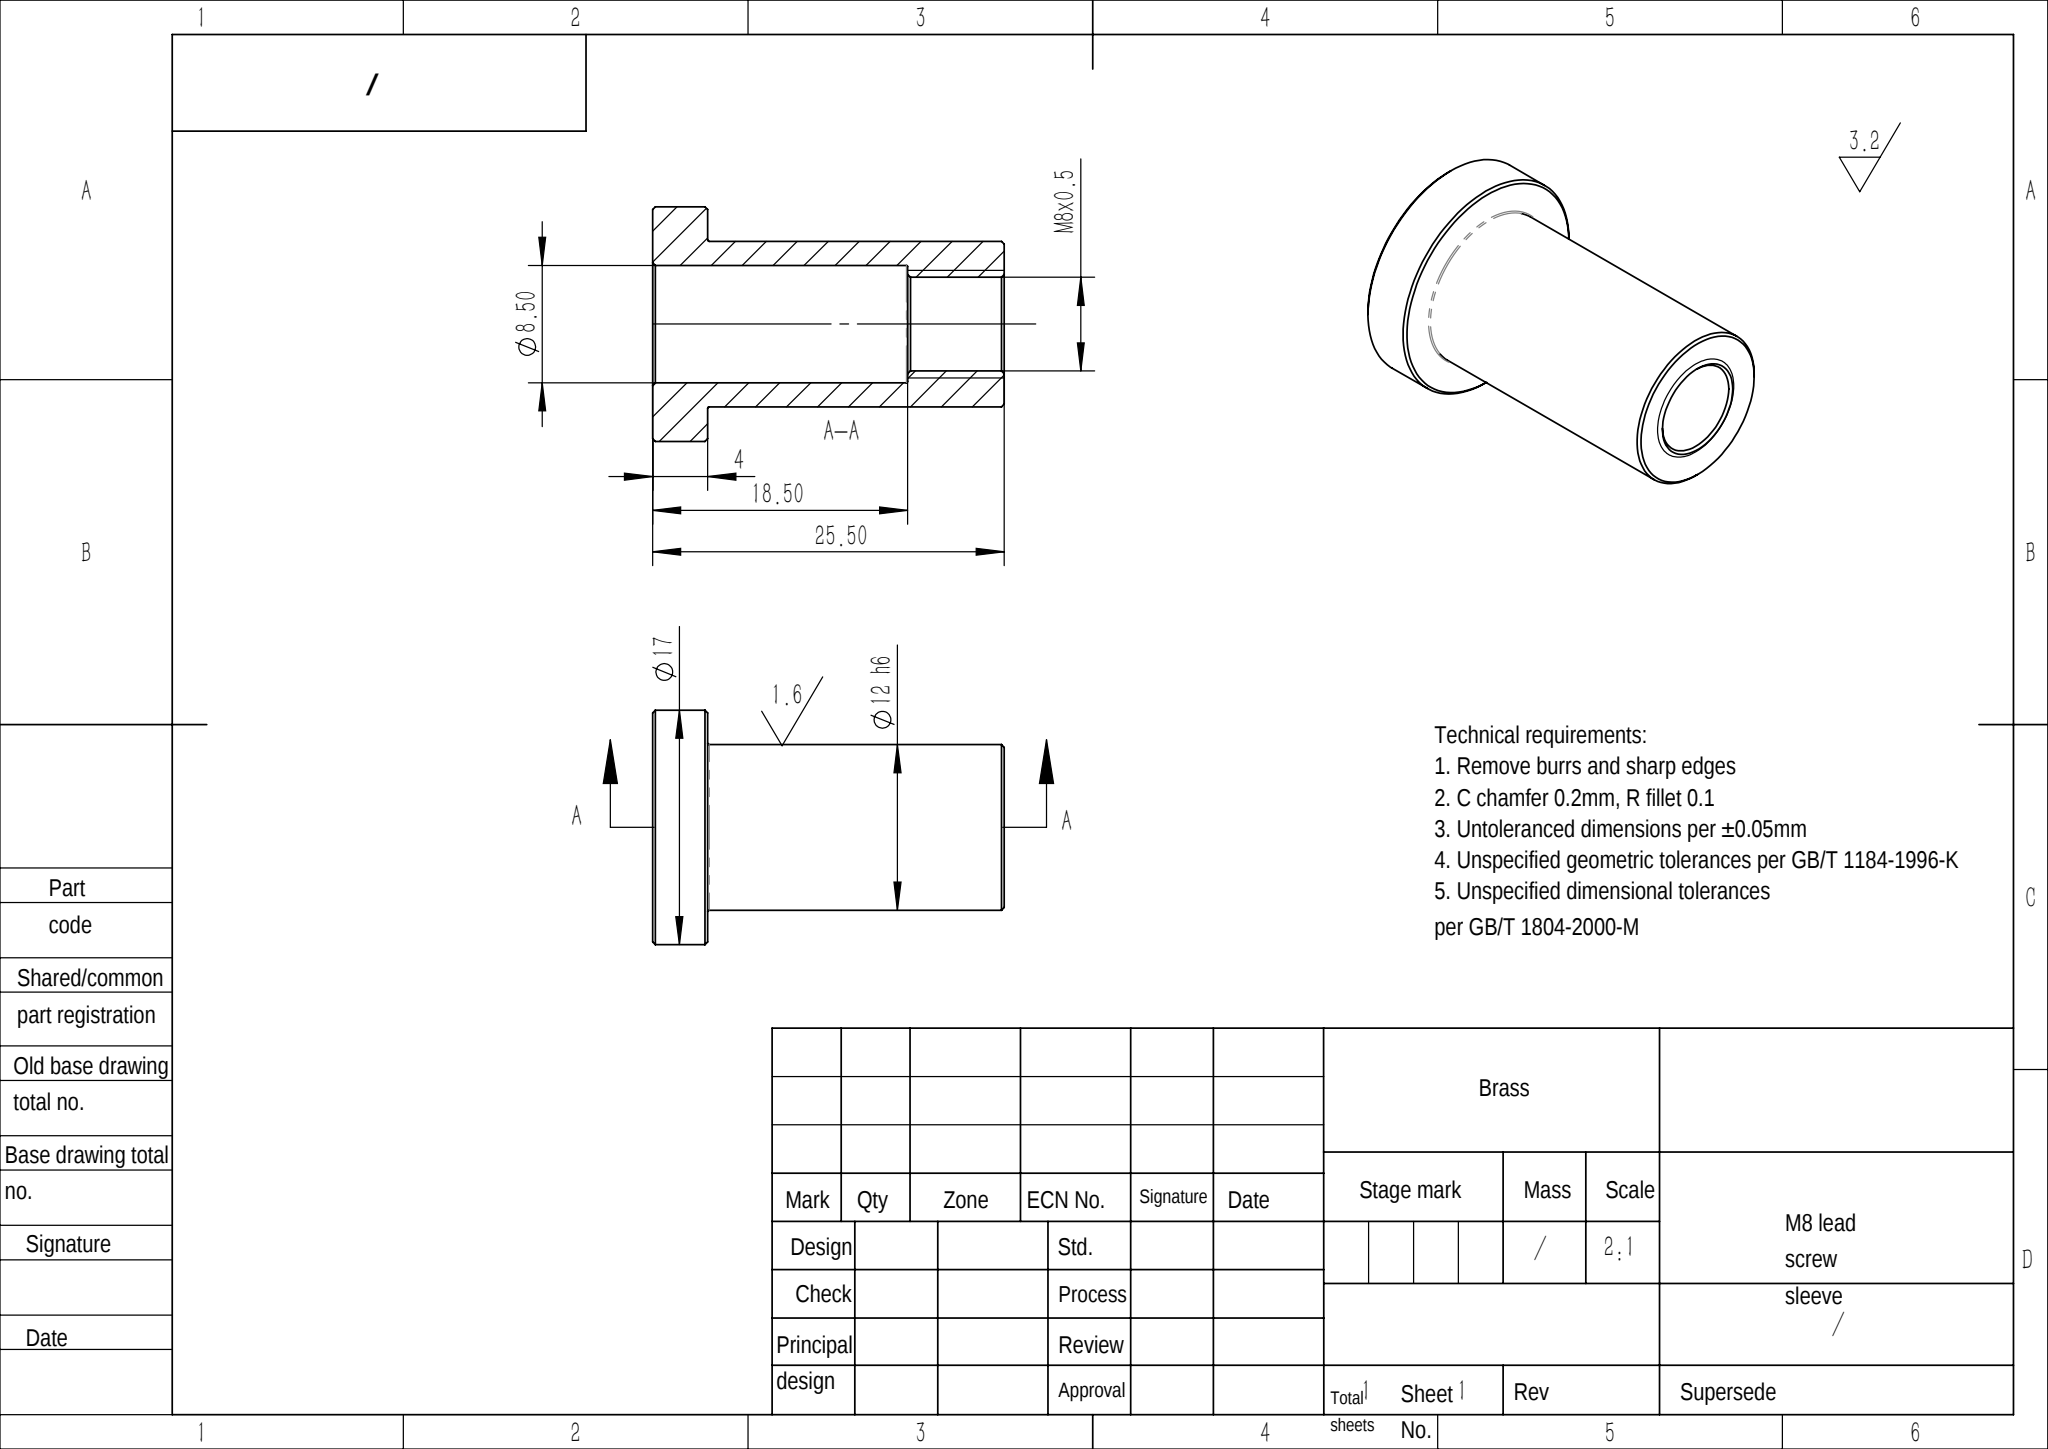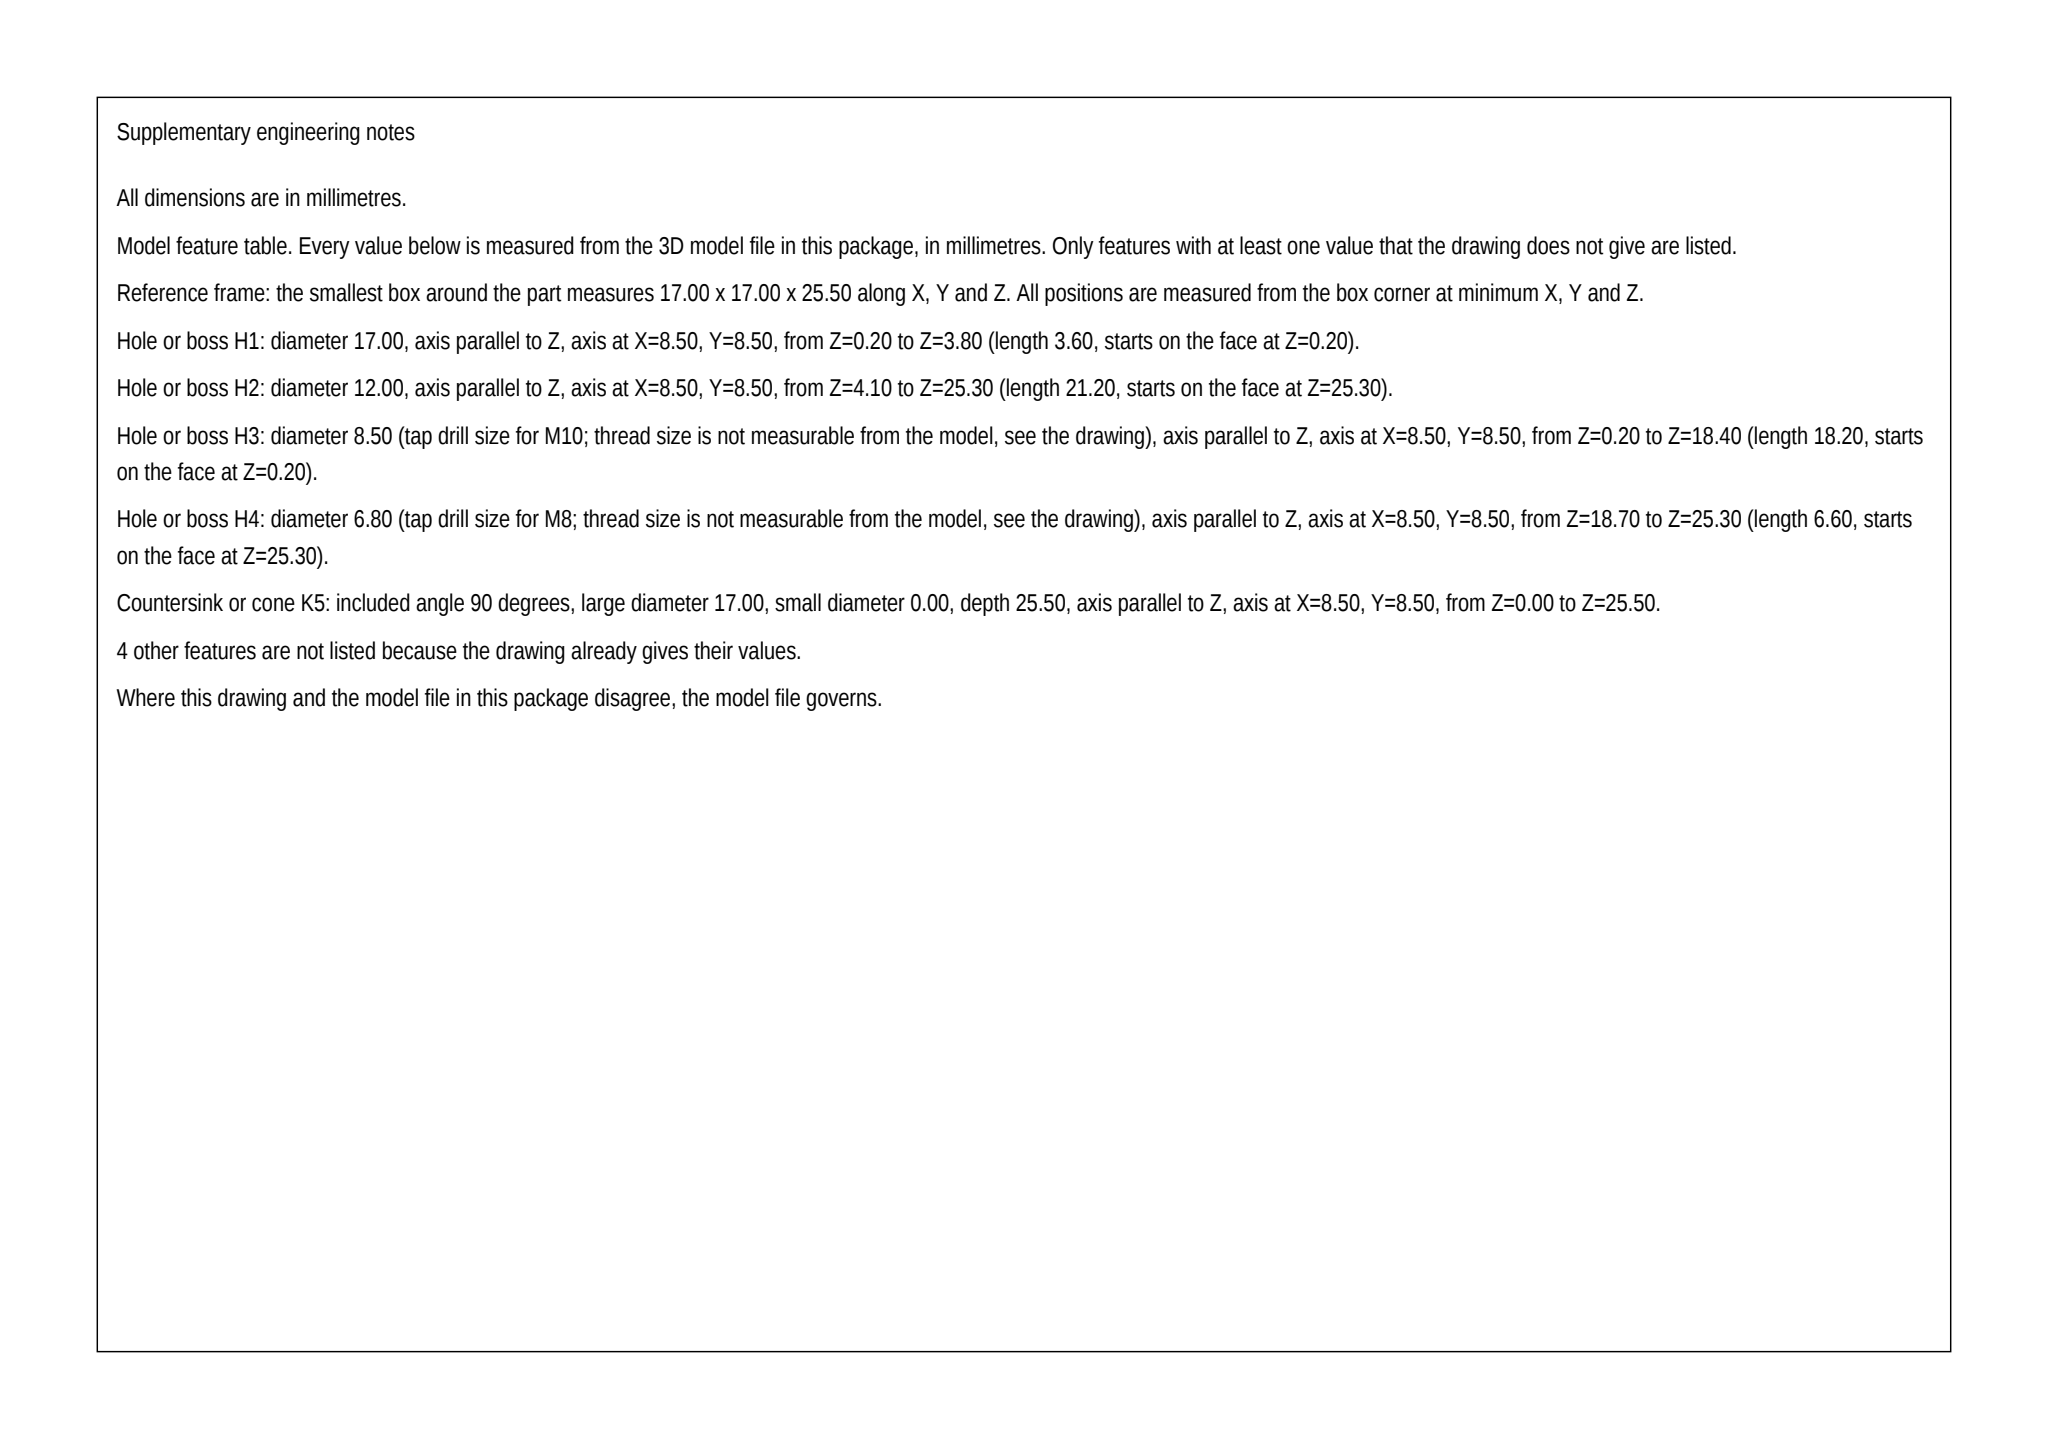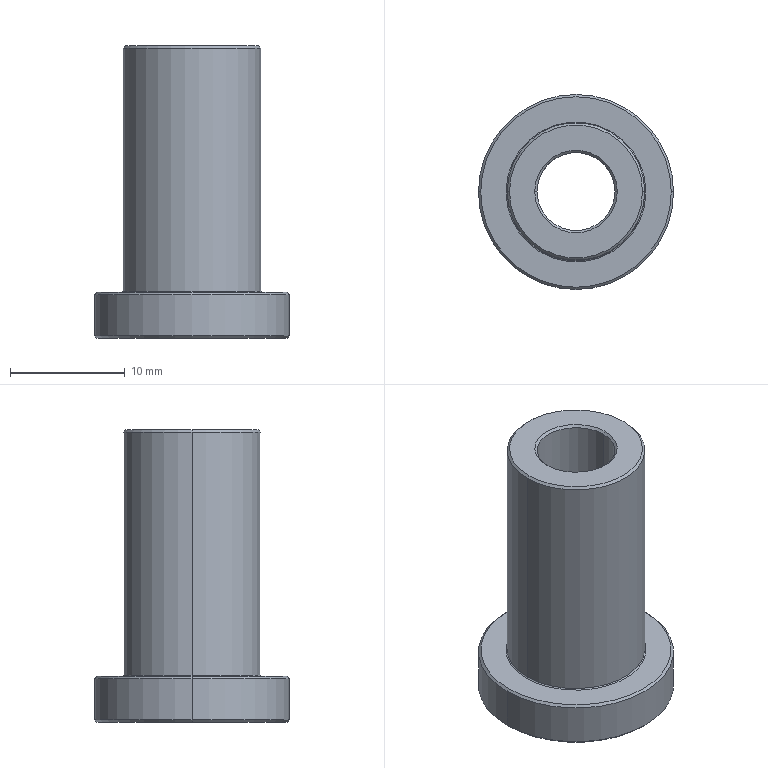Part | SolidWorks | mm | material Brass | 1 solid | 28 faces | box 17 x 17 x 25.5 mm | volume 2031 mm3 | cone 12 | cylinder 8 | torus 4 | plane 4 | commonest cylinder face diameters 6.8 x2 12 x2 8.5 x2 17 x2
STEP:
#1=CARTESIAN_POINT('',(-4.25,0.,18.4));
#2=VERTEX_POINT('',#1);
#3=CARTESIAN_POINT('',(4.25,0.,18.4));
#4=VERTEX_POINT('',#3);
#5=CARTESIAN_POINT('',(0.,0.,18.4));
#6=DIRECTION('',(0.,0.,1.));
#7=DIRECTION('',(1.,0.,0.));
#8=AXIS2_PLACEMENT_3D('',#5,#6,#7);
#9=CIRCLE('',#8,4.25);
#10=EDGE_CURVE('',#2,#4,#9,.T.);
#11=ORIENTED_EDGE('',*,*,#10,.F.);
#12=CARTESIAN_POINT('',(-4.15,0.,18.5));
#13=VERTEX_POINT('',#12);
#14=CARTESIAN_POINT('',(-4.15,0.,18.4));
#15=DIRECTION('',(0.,1.,0.));
#16=DIRECTION('',(-1.,0.,0.));
#17=AXIS2_PLACEMENT_3D('',#14,#15,#16);
#18=CIRCLE('',#17,0.1);
#19=EDGE_CURVE('',#2,#13,#18,.T.);
#20=ORIENTED_EDGE('',*,*,#19,.T.);
#21=CARTESIAN_POINT('',(4.15,0.,18.5));
#22=VERTEX_POINT('',#21);
#23=CARTESIAN_POINT('',(0.,0.,18.5));
#24=DIRECTION('',(0.,0.,-1.));
#25=DIRECTION('',(1.,0.,0.));
#26=AXIS2_PLACEMENT_3D('',#23,#24,#25);
#27=CIRCLE('',#26,4.15);
#28=EDGE_CURVE('',#22,#13,#27,.T.);
#29=ORIENTED_EDGE('',*,*,#28,.F.);
#30=CARTESIAN_POINT('',(4.15,0.,18.4));
#31=DIRECTION('',(0.,-1.,0.));
#32=DIRECTION('',(0.,0.,-1.));
#33=AXIS2_PLACEMENT_3D('',#30,#31,#32);
#34=CIRCLE('',#33,0.1);
#35=EDGE_CURVE('',#4,#22,#34,.T.);
#36=ORIENTED_EDGE('',*,*,#35,.F.);
#37=EDGE_LOOP('',(#11,#20,#29,#36));
#38=FACE_OUTER_BOUND('',#37,.T.);
#39=CARTESIAN_POINT('',(0.,0.,18.4));
#40=DIRECTION('',(0.,0.,1.));
#41=DIRECTION('',(1.,0.,0.));
#42=AXIS2_PLACEMENT_3D('',#39,#40,#41);
#43=TOROIDAL_SURFACE('',#42,4.15,0.1);
#44=ADVANCED_FACE('',(#38),#43,.F.);
#45=CARTESIAN_POINT('',(-6.,0.,4.1));
#46=VERTEX_POINT('',#45);
#47=CARTESIAN_POINT('',(6.,0.,4.1));
#48=VERTEX_POINT('',#47);
#49=CARTESIAN_POINT('',(0.,0.,4.1));
#50=DIRECTION('',(0.,0.,1.));
#51=DIRECTION('',(1.,0.,0.));
#52=AXIS2_PLACEMENT_3D('',#49,#50,#51);
#53=CIRCLE('',#52,6.);
#54=EDGE_CURVE('',#46,#48,#53,.T.);
#55=ORIENTED_EDGE('',*,*,#54,.F.);
#56=CARTESIAN_POINT('',(-6.1,0.,4.));
#57=VERTEX_POINT('',#56);
#58=CARTESIAN_POINT('',(-6.1,0.,4.1));
#59=DIRECTION('',(0.,1.,0.));
#60=DIRECTION('',(-1.,0.,0.));
#61=AXIS2_PLACEMENT_3D('',#58,#59,#60);
#62=CIRCLE('',#61,0.1);
#63=EDGE_CURVE('',#46,#57,#62,.T.);
#64=ORIENTED_EDGE('',*,*,#63,.T.);
#65=CARTESIAN_POINT('',(6.1,0.,4.));
#66=VERTEX_POINT('',#65);
#67=CARTESIAN_POINT('',(0.,0.,4.));
#68=DIRECTION('',(0.,0.,-1.));
#69=DIRECTION('',(1.,0.,0.));
#70=AXIS2_PLACEMENT_3D('',#67,#68,#69);
#71=CIRCLE('',#70,6.1);
#72=EDGE_CURVE('',#66,#57,#71,.T.);
#73=ORIENTED_EDGE('',*,*,#72,.F.);
#74=CARTESIAN_POINT('',(6.1,0.,4.1));
#75=DIRECTION('',(0.,-1.,0.));
#76=DIRECTION('',(0.,0.,-1.));
#77=AXIS2_PLACEMENT_3D('',#74,#75,#76);
#78=CIRCLE('',#77,0.1);
#79=EDGE_CURVE('',#48,#66,#78,.T.);
#80=ORIENTED_EDGE('',*,*,#79,.F.);
#81=EDGE_LOOP('',(#55,#64,#73,#80));
#82=FACE_OUTER_BOUND('',#81,.T.);
#83=CARTESIAN_POINT('',(0.,0.,4.1));
#84=DIRECTION('',(0.,0.,1.));
#85=DIRECTION('',(1.,0.,0.));
#86=AXIS2_PLACEMENT_3D('',#83,#84,#85);
#87=TOROIDAL_SURFACE('',#86,6.1,0.1);
#88=ADVANCED_FACE('',(#82),#87,.F.);
#89=CARTESIAN_POINT('',(8.3,0.,4.));
#90=VERTEX_POINT('',#89);
#91=CARTESIAN_POINT('',(-8.3,0.,4.));
#92=VERTEX_POINT('',#91);
#93=CARTESIAN_POINT('',(0.,0.,4.));
#94=DIRECTION('',(0.,0.,1.));
#95=DIRECTION('',(1.,0.,0.));
#96=AXIS2_PLACEMENT_3D('',#93,#94,#95);
#97=CIRCLE('',#96,8.3);
#98=EDGE_CURVE('',#90,#92,#97,.T.);
#99=ORIENTED_EDGE('',*,*,#98,.F.);
#100=CARTESIAN_POINT('',(8.5,0.,3.8));
#101=VERTEX_POINT('',#100);
#102=CARTESIAN_POINT('',(8.3,0.,4.));
#103=DIRECTION('',(0.7071,0.,-0.7071));
#104=VECTOR('',#103,1000.);
#105=LINE('',#102,#104);
#106=EDGE_CURVE('',#90,#101,#105,.T.);
#107=ORIENTED_EDGE('',*,*,#106,.T.);
#108=CARTESIAN_POINT('',(-8.5,0.,3.8));
#109=VERTEX_POINT('',#108);
#110=CARTESIAN_POINT('',(0.,0.,3.8));
#111=DIRECTION('',(0.,0.,-1.));
#112=DIRECTION('',(1.,0.,0.));
#113=AXIS2_PLACEMENT_3D('',#110,#111,#112);
#114=CIRCLE('',#113,8.5);
#115=EDGE_CURVE('',#109,#101,#114,.T.);
#116=ORIENTED_EDGE('',*,*,#115,.F.);
#117=CARTESIAN_POINT('',(-8.3,0.,4.));
#118=DIRECTION('',(-0.7071,0.,-0.7071));
#119=VECTOR('',#118,1000.);
#120=LINE('',#117,#119);
#121=EDGE_CURVE('',#92,#109,#120,.T.);
#122=ORIENTED_EDGE('',*,*,#121,.F.);
#123=EDGE_LOOP('',(#99,#107,#116,#122));
#124=FACE_OUTER_BOUND('',#123,.T.);
#125=CARTESIAN_POINT('',(0.,0.,4.));
#126=DIRECTION('',(0.,0.,-1.));
#127=DIRECTION('',(-1.,0.,0.));
#128=AXIS2_PLACEMENT_3D('',#125,#126,#127);
#129=CONICAL_SURFACE('',#128,8.3,0.7854);
#130=ADVANCED_FACE('',(#124),#129,.T.);
#131=CARTESIAN_POINT('',(3.4,0.,18.7));
#132=VERTEX_POINT('',#131);
#133=CARTESIAN_POINT('',(-3.4,0.,18.7));
#134=VERTEX_POINT('',#133);
#135=CARTESIAN_POINT('',(0.,0.,18.7));
#136=DIRECTION('',(0.,0.,-1.));
#137=DIRECTION('',(1.,0.,0.));
#138=AXIS2_PLACEMENT_3D('',#135,#136,#137);
#139=CIRCLE('',#138,3.4);
#140=EDGE_CURVE('',#132,#134,#139,.T.);
#141=ORIENTED_EDGE('',*,*,#140,.F.);
#142=CARTESIAN_POINT('',(3.6,0.,18.5));
#143=VERTEX_POINT('',#142);
#144=CARTESIAN_POINT('',(3.6,0.,18.5));
#145=DIRECTION('',(0.7071,0.,-0.7071));
#146=VECTOR('',#145,1000.);
#147=LINE('',#144,#146);
#148=EDGE_CURVE('',#132,#143,#147,.T.);
#149=ORIENTED_EDGE('',*,*,#148,.T.);
#150=CARTESIAN_POINT('',(-3.6,0.,18.5));
#151=VERTEX_POINT('',#150);
#152=CARTESIAN_POINT('',(0.,0.,18.5));
#153=DIRECTION('',(0.,0.,1.));
#154=DIRECTION('',(1.,0.,0.));
#155=AXIS2_PLACEMENT_3D('',#152,#153,#154);
#156=CIRCLE('',#155,3.6);
#157=EDGE_CURVE('',#151,#143,#156,.T.);
#158=ORIENTED_EDGE('',*,*,#157,.F.);
#159=CARTESIAN_POINT('',(-3.6,0.,18.5));
#160=DIRECTION('',(-0.7071,0.,-0.7071));
#161=VECTOR('',#160,1000.);
#162=LINE('',#159,#161);
#163=EDGE_CURVE('',#134,#151,#162,.T.);
#164=ORIENTED_EDGE('',*,*,#163,.F.);
#165=EDGE_LOOP('',(#141,#149,#158,#164));
#166=FACE_OUTER_BOUND('',#165,.T.);
#167=CARTESIAN_POINT('',(0.,0.,18.5));
#168=DIRECTION('',(0.,0.,-1.));
#169=DIRECTION('',(-1.,0.,0.));
#170=AXIS2_PLACEMENT_3D('',#167,#168,#169);
#171=CONICAL_SURFACE('',#170,3.6,0.7854);
#172=ADVANCED_FACE('',(#166),#171,.F.);
#173=CARTESIAN_POINT('',(-8.3,0.,0.));
#174=VERTEX_POINT('',#173);
#175=CARTESIAN_POINT('',(8.3,0.,0.));
#176=VERTEX_POINT('',#175);
#177=CARTESIAN_POINT('',(0.,0.,0.));
#178=DIRECTION('',(0.,0.,-1.));
#179=DIRECTION('',(1.,0.,0.));
#180=AXIS2_PLACEMENT_3D('',#177,#178,#179);
#181=CIRCLE('',#180,8.3);
#182=EDGE_CURVE('',#174,#176,#181,.T.);
#183=ORIENTED_EDGE('',*,*,#182,.F.);
#184=CARTESIAN_POINT('',(-8.5,0.,0.2));
#185=VERTEX_POINT('',#184);
#186=CARTESIAN_POINT('',(-8.5,0.,0.2));
#187=DIRECTION('',(-0.7071,0.,0.7071));
#188=VECTOR('',#187,1000.);
#189=LINE('',#186,#188);
#190=EDGE_CURVE('',#174,#185,#189,.T.);
#191=ORIENTED_EDGE('',*,*,#190,.T.);
#192=CARTESIAN_POINT('',(8.5,0.,0.2));
#193=VERTEX_POINT('',#192);
#194=CARTESIAN_POINT('',(0.,0.,0.2));
#195=DIRECTION('',(0.,0.,1.));
#196=DIRECTION('',(1.,0.,0.));
#197=AXIS2_PLACEMENT_3D('',#194,#195,#196);
#198=CIRCLE('',#197,8.5);
#199=EDGE_CURVE('',#193,#185,#198,.T.);
#200=ORIENTED_EDGE('',*,*,#199,.F.);
#201=CARTESIAN_POINT('',(8.5,0.,0.2));
#202=DIRECTION('',(0.7071,0.,0.7071));
#203=VECTOR('',#202,1000.);
#204=LINE('',#201,#203);
#205=EDGE_CURVE('',#176,#193,#204,.T.);
#206=ORIENTED_EDGE('',*,*,#205,.F.);
#207=EDGE_LOOP('',(#183,#191,#200,#206));
#208=FACE_OUTER_BOUND('',#207,.T.);
#209=CARTESIAN_POINT('',(0.,0.,0.2));
#210=DIRECTION('',(0.,0.,1.));
#211=DIRECTION('',(1.,0.,0.));
#212=AXIS2_PLACEMENT_3D('',#209,#210,#211);
#213=CONICAL_SURFACE('',#212,8.5,0.7854);
#214=ADVANCED_FACE('',(#208),#213,.T.);
#215=CARTESIAN_POINT('',(4.25,0.,0.2));
#216=VERTEX_POINT('',#215);
#217=CARTESIAN_POINT('',(-4.25,0.,0.2));
#218=VERTEX_POINT('',#217);
#219=CARTESIAN_POINT('',(0.,0.,0.2));
#220=DIRECTION('',(0.,0.,-1.));
#221=DIRECTION('',(1.,0.,0.));
#222=AXIS2_PLACEMENT_3D('',#219,#220,#221);
#223=CIRCLE('',#222,4.25);
#224=EDGE_CURVE('',#216,#218,#223,.T.);
#225=ORIENTED_EDGE('',*,*,#224,.F.);
#226=CARTESIAN_POINT('',(4.45,0.,0.));
#227=VERTEX_POINT('',#226);
#228=CARTESIAN_POINT('',(4.45,0.,0.));
#229=DIRECTION('',(0.7071,0.,-0.7071));
#230=VECTOR('',#229,1000.);
#231=LINE('',#228,#230);
#232=EDGE_CURVE('',#216,#227,#231,.T.);
#233=ORIENTED_EDGE('',*,*,#232,.T.);
#234=CARTESIAN_POINT('',(-4.45,0.,0.));
#235=VERTEX_POINT('',#234);
#236=CARTESIAN_POINT('',(0.,0.,0.));
#237=DIRECTION('',(0.,0.,1.));
#238=DIRECTION('',(1.,0.,0.));
#239=AXIS2_PLACEMENT_3D('',#236,#237,#238);
#240=CIRCLE('',#239,4.45);
#241=EDGE_CURVE('',#235,#227,#240,.T.);
#242=ORIENTED_EDGE('',*,*,#241,.F.);
#243=CARTESIAN_POINT('',(-4.45,0.,0.));
#244=DIRECTION('',(-0.7071,0.,-0.7071));
#245=VECTOR('',#244,1000.);
#246=LINE('',#243,#245);
#247=EDGE_CURVE('',#218,#235,#246,.T.);
#248=ORIENTED_EDGE('',*,*,#247,.F.);
#249=EDGE_LOOP('',(#225,#233,#242,#248));
#250=FACE_OUTER_BOUND('',#249,.T.);
#251=CARTESIAN_POINT('',(0.,0.,0.));
#252=DIRECTION('',(0.,0.,-1.));
#253=DIRECTION('',(-1.,0.,0.));
#254=AXIS2_PLACEMENT_3D('',#251,#252,#253);
#255=CONICAL_SURFACE('',#254,4.45,0.7854);
#256=ADVANCED_FACE('',(#250),#255,.F.);
#257=CARTESIAN_POINT('',(5.8,0.,25.5));
#258=VERTEX_POINT('',#257);
#259=CARTESIAN_POINT('',(-5.8,0.,25.5));
#260=VERTEX_POINT('',#259);
#261=CARTESIAN_POINT('',(0.,0.,25.5));
#262=DIRECTION('',(0.,0.,1.));
#263=DIRECTION('',(1.,0.,0.));
#264=AXIS2_PLACEMENT_3D('',#261,#262,#263);
#265=CIRCLE('',#264,5.8);
#266=EDGE_CURVE('',#258,#260,#265,.T.);
#267=ORIENTED_EDGE('',*,*,#266,.F.);
#268=CARTESIAN_POINT('',(6.,0.,25.3));
#269=VERTEX_POINT('',#268);
#270=CARTESIAN_POINT('',(5.8,0.,25.5));
#271=DIRECTION('',(0.7071,0.,-0.7071));
#272=VECTOR('',#271,1000.);
#273=LINE('',#270,#272);
#274=EDGE_CURVE('',#258,#269,#273,.T.);
#275=ORIENTED_EDGE('',*,*,#274,.T.);
#276=CARTESIAN_POINT('',(-6.,0.,25.3));
#277=VERTEX_POINT('',#276);
#278=CARTESIAN_POINT('',(0.,0.,25.3));
#279=DIRECTION('',(0.,0.,-1.));
#280=DIRECTION('',(1.,0.,0.));
#281=AXIS2_PLACEMENT_3D('',#278,#279,#280);
#282=CIRCLE('',#281,6.);
#283=EDGE_CURVE('',#277,#269,#282,.T.);
#284=ORIENTED_EDGE('',*,*,#283,.F.);
#285=CARTESIAN_POINT('',(-5.8,0.,25.5));
#286=DIRECTION('',(-0.7071,0.,-0.7071));
#287=VECTOR('',#286,1000.);
#288=LINE('',#285,#287);
#289=EDGE_CURVE('',#260,#277,#288,.T.);
#290=ORIENTED_EDGE('',*,*,#289,.F.);
#291=EDGE_LOOP('',(#267,#275,#284,#290));
#292=FACE_OUTER_BOUND('',#291,.T.);
#293=CARTESIAN_POINT('',(0.,0.,25.5));
#294=DIRECTION('',(0.,0.,-1.));
#295=DIRECTION('',(-1.,0.,0.));
#296=AXIS2_PLACEMENT_3D('',#293,#294,#295);
#297=CONICAL_SURFACE('',#296,5.8,0.7854);
#298=ADVANCED_FACE('',(#292),#297,.T.);
#299=CARTESIAN_POINT('',(-3.4,0.,25.3));
#300=VERTEX_POINT('',#299);
#301=CARTESIAN_POINT('',(3.4,0.,25.3));
#302=VERTEX_POINT('',#301);
#303=CARTESIAN_POINT('',(0.,0.,25.3));
#304=DIRECTION('',(0.,0.,1.));
#305=DIRECTION('',(1.,0.,0.));
#306=AXIS2_PLACEMENT_3D('',#303,#304,#305);
#307=CIRCLE('',#306,3.4);
#308=EDGE_CURVE('',#300,#302,#307,.T.);
#309=ORIENTED_EDGE('',*,*,#308,.F.);
#310=CARTESIAN_POINT('',(-3.6,0.,25.5));
#311=VERTEX_POINT('',#310);
#312=CARTESIAN_POINT('',(-3.4,0.,25.3));
#313=DIRECTION('',(-0.7071,0.,0.7071));
#314=VECTOR('',#313,1000.);
#315=LINE('',#312,#314);
#316=EDGE_CURVE('',#300,#311,#315,.T.);
#317=ORIENTED_EDGE('',*,*,#316,.T.);
#318=CARTESIAN_POINT('',(3.6,0.,25.5));
#319=VERTEX_POINT('',#318);
#320=CARTESIAN_POINT('',(0.,0.,25.5));
#321=DIRECTION('',(0.,0.,-1.));
#322=DIRECTION('',(1.,0.,0.));
#323=AXIS2_PLACEMENT_3D('',#320,#321,#322);
#324=CIRCLE('',#323,3.6);
#325=EDGE_CURVE('',#319,#311,#324,.T.);
#326=ORIENTED_EDGE('',*,*,#325,.F.);
#327=CARTESIAN_POINT('',(3.4,0.,25.3));
#328=DIRECTION('',(0.7071,0.,0.7071));
#329=VECTOR('',#328,1000.);
#330=LINE('',#327,#329);
#331=EDGE_CURVE('',#302,#319,#330,.T.);
#332=ORIENTED_EDGE('',*,*,#331,.F.);
#333=EDGE_LOOP('',(#309,#317,#326,#332));
#334=FACE_OUTER_BOUND('',#333,.T.);
#335=CARTESIAN_POINT('',(0.,0.,25.3));
#336=DIRECTION('',(0.,0.,1.));
#337=DIRECTION('',(1.,0.,0.));
#338=AXIS2_PLACEMENT_3D('',#335,#336,#337);
#339=CONICAL_SURFACE('',#338,3.4,0.7854);
#340=ADVANCED_FACE('',(#334),#339,.F.);
#341=ORIENTED_EDGE('',*,*,#308,.T.);
#342=CARTESIAN_POINT('',(3.4,0.,30.));
#343=DIRECTION('',(0.,0.,-1.));
#344=VECTOR('',#343,1000.);
#345=LINE('',#342,#344);
#346=EDGE_CURVE('',#302,#132,#345,.T.);
#347=ORIENTED_EDGE('',*,*,#346,.T.);
#348=ORIENTED_EDGE('',*,*,#140,.T.);
#349=CARTESIAN_POINT('',(-3.4,0.,30.));
#350=DIRECTION('',(0.,0.,-1.));
#351=VECTOR('',#350,1000.);
#352=LINE('',#349,#351);
#353=EDGE_CURVE('',#300,#134,#352,.T.);
#354=ORIENTED_EDGE('',*,*,#353,.F.);
#355=EDGE_LOOP('',(#341,#347,#348,#354));
#356=FACE_OUTER_BOUND('',#355,.T.);
#357=CARTESIAN_POINT('',(0.,0.,30.));
#358=DIRECTION('',(0.,0.,-1.));
#359=DIRECTION('',(-1.,0.,0.));
#360=AXIS2_PLACEMENT_3D('',#357,#358,#359);
#361=CYLINDRICAL_SURFACE('',#360,3.4);
#362=ADVANCED_FACE('',(#356),#361,.F.);
#363=CARTESIAN_POINT('',(0.,0.,4.1));
#364=DIRECTION('',(0.,0.,1.));
#365=DIRECTION('',(1.,0.,0.));
#366=AXIS2_PLACEMENT_3D('',#363,#364,#365);
#367=CIRCLE('',#366,6.);
#368=EDGE_CURVE('',#48,#46,#367,.T.);
#369=ORIENTED_EDGE('',*,*,#368,.T.);
#370=CARTESIAN_POINT('',(-6.,0.,4.));
#371=DIRECTION('',(0.,0.,1.));
#372=VECTOR('',#371,1000.);
#373=LINE('',#370,#372);
#374=EDGE_CURVE('',#46,#277,#373,.T.);
#375=ORIENTED_EDGE('',*,*,#374,.T.);
#376=ORIENTED_EDGE('',*,*,#283,.T.);
#377=CARTESIAN_POINT('',(6.,0.,4.));
#378=DIRECTION('',(0.,0.,1.));
#379=VECTOR('',#378,1000.);
#380=LINE('',#377,#379);
#381=EDGE_CURVE('',#48,#269,#380,.T.);
#382=ORIENTED_EDGE('',*,*,#381,.F.);
#383=EDGE_LOOP('',(#369,#375,#376,#382));
#384=FACE_OUTER_BOUND('',#383,.T.);
#385=CARTESIAN_POINT('',(0.,0.,4.));
#386=DIRECTION('',(0.,0.,1.));
#387=DIRECTION('',(1.,0.,0.));
#388=AXIS2_PLACEMENT_3D('',#385,#386,#387);
#389=CYLINDRICAL_SURFACE('',#388,6.);
#390=ADVANCED_FACE('',(#384),#389,.T.);
#391=ORIENTED_EDGE('',*,*,#10,.T.);
#392=CARTESIAN_POINT('',(4.25,0.,18.5));
#393=DIRECTION('',(0.,0.,-1.));
#394=VECTOR('',#393,1000.);
#395=LINE('',#392,#394);
#396=EDGE_CURVE('',#4,#216,#395,.T.);
#397=ORIENTED_EDGE('',*,*,#396,.T.);
#398=ORIENTED_EDGE('',*,*,#224,.T.);
#399=CARTESIAN_POINT('',(-4.25,0.,18.5));
#400=DIRECTION('',(0.,0.,-1.));
#401=VECTOR('',#400,1000.);
#402=LINE('',#399,#401);
#403=EDGE_CURVE('',#2,#218,#402,.T.);
#404=ORIENTED_EDGE('',*,*,#403,.F.);
#405=EDGE_LOOP('',(#391,#397,#398,#404));
#406=FACE_OUTER_BOUND('',#405,.T.);
#407=CARTESIAN_POINT('',(0.,0.,18.5));
#408=DIRECTION('',(0.,0.,-1.));
#409=DIRECTION('',(-1.,0.,0.));
#410=AXIS2_PLACEMENT_3D('',#407,#408,#409);
#411=CYLINDRICAL_SURFACE('',#410,4.25);
#412=ADVANCED_FACE('',(#406),#411,.F.);
#413=ORIENTED_EDGE('',*,*,#115,.T.);
#414=CARTESIAN_POINT('',(8.5,0.,18.5));
#415=DIRECTION('',(0.,0.,-1.));
#416=VECTOR('',#415,1000.);
#417=LINE('',#414,#416);
#418=EDGE_CURVE('',#101,#193,#417,.T.);
#419=ORIENTED_EDGE('',*,*,#418,.T.);
#420=ORIENTED_EDGE('',*,*,#199,.T.);
#421=CARTESIAN_POINT('',(-8.5,0.,18.5));
#422=DIRECTION('',(0.,0.,-1.));
#423=VECTOR('',#422,1000.);
#424=LINE('',#421,#423);
#425=EDGE_CURVE('',#109,#185,#424,.T.);
#426=ORIENTED_EDGE('',*,*,#425,.F.);
#427=EDGE_LOOP('',(#413,#419,#420,#426));
#428=FACE_OUTER_BOUND('',#427,.T.);
#429=CARTESIAN_POINT('',(0.,0.,18.5));
#430=DIRECTION('',(0.,0.,-1.));
#431=DIRECTION('',(-1.,0.,0.));
#432=AXIS2_PLACEMENT_3D('',#429,#430,#431);
#433=CYLINDRICAL_SURFACE('',#432,8.5);
#434=ADVANCED_FACE('',(#428),#433,.T.);
#435=ORIENTED_EDGE('',*,*,#418,.F.);
#436=CARTESIAN_POINT('',(0.,0.,3.8));
#437=DIRECTION('',(0.,0.,-1.));
#438=DIRECTION('',(1.,0.,0.));
#439=AXIS2_PLACEMENT_3D('',#436,#437,#438);
#440=CIRCLE('',#439,8.5);
#441=EDGE_CURVE('',#101,#109,#440,.T.);
#442=ORIENTED_EDGE('',*,*,#441,.T.);
#443=ORIENTED_EDGE('',*,*,#425,.T.);
#444=CARTESIAN_POINT('',(0.,0.,0.2));
#445=DIRECTION('',(0.,0.,1.));
#446=DIRECTION('',(1.,0.,0.));
#447=AXIS2_PLACEMENT_3D('',#444,#445,#446);
#448=CIRCLE('',#447,8.5);
#449=EDGE_CURVE('',#185,#193,#448,.T.);
#450=ORIENTED_EDGE('',*,*,#449,.T.);
#451=EDGE_LOOP('',(#435,#442,#443,#450));
#452=FACE_OUTER_BOUND('',#451,.T.);
#453=CARTESIAN_POINT('',(0.,0.,18.5));
#454=DIRECTION('',(0.,0.,-1.));
#455=DIRECTION('',(-1.,0.,0.));
#456=AXIS2_PLACEMENT_3D('',#453,#454,#455);
#457=CYLINDRICAL_SURFACE('',#456,8.5);
#458=ADVANCED_FACE('',(#452),#457,.T.);
#459=ORIENTED_EDGE('',*,*,#241,.T.);
#460=CARTESIAN_POINT('',(0.,0.,0.));
#461=DIRECTION('',(0.,0.,1.));
#462=DIRECTION('',(1.,0.,0.));
#463=AXIS2_PLACEMENT_3D('',#460,#461,#462);
#464=CIRCLE('',#463,4.45);
#465=EDGE_CURVE('',#227,#235,#464,.T.);
#466=ORIENTED_EDGE('',*,*,#465,.T.);
#467=EDGE_LOOP('',(#459,#466));
#468=FACE_BOUND('',#467,.T.);
#469=CARTESIAN_POINT('',(0.,0.,0.));
#470=DIRECTION('',(0.,0.,-1.));
#471=DIRECTION('',(1.,0.,0.));
#472=AXIS2_PLACEMENT_3D('',#469,#470,#471);
#473=CIRCLE('',#472,8.3);
#474=EDGE_CURVE('',#176,#174,#473,.T.);
#475=ORIENTED_EDGE('',*,*,#474,.T.);
#476=ORIENTED_EDGE('',*,*,#182,.T.);
#477=EDGE_LOOP('',(#475,#476));
#478=FACE_OUTER_BOUND('',#477,.T.);
#479=CARTESIAN_POINT('',(0.,0.,0.));
#480=DIRECTION('',(0.,0.,1.));
#481=DIRECTION('',(1.,0.,0.));
#482=AXIS2_PLACEMENT_3D('',#479,#480,#481);
#483=PLANE('',#482);
#484=ADVANCED_FACE('',(#468,#478),#483,.F.);
#485=ORIENTED_EDGE('',*,*,#396,.F.);
#486=CARTESIAN_POINT('',(0.,0.,18.4));
#487=DIRECTION('',(0.,0.,1.));
#488=DIRECTION('',(1.,0.,0.));
#489=AXIS2_PLACEMENT_3D('',#486,#487,#488);
#490=CIRCLE('',#489,4.25);
#491=EDGE_CURVE('',#4,#2,#490,.T.);
#492=ORIENTED_EDGE('',*,*,#491,.T.);
#493=ORIENTED_EDGE('',*,*,#403,.T.);
#494=CARTESIAN_POINT('',(0.,0.,0.2));
#495=DIRECTION('',(0.,0.,-1.));
#496=DIRECTION('',(1.,0.,0.));
#497=AXIS2_PLACEMENT_3D('',#494,#495,#496);
#498=CIRCLE('',#497,4.25);
#499=EDGE_CURVE('',#218,#216,#498,.T.);
#500=ORIENTED_EDGE('',*,*,#499,.T.);
#501=EDGE_LOOP('',(#485,#492,#493,#500));
#502=FACE_OUTER_BOUND('',#501,.T.);
#503=CARTESIAN_POINT('',(0.,0.,18.5));
#504=DIRECTION('',(0.,0.,-1.));
#505=DIRECTION('',(-1.,0.,0.));
#506=AXIS2_PLACEMENT_3D('',#503,#504,#505);
#507=CYLINDRICAL_SURFACE('',#506,4.25);
#508=ADVANCED_FACE('',(#502),#507,.F.);
#509=ORIENTED_EDGE('',*,*,#72,.T.);
#510=CARTESIAN_POINT('',(0.,0.,4.));
#511=DIRECTION('',(0.,0.,-1.));
#512=DIRECTION('',(1.,0.,0.));
#513=AXIS2_PLACEMENT_3D('',#510,#511,#512);
#514=CIRCLE('',#513,6.1);
#515=EDGE_CURVE('',#57,#66,#514,.T.);
#516=ORIENTED_EDGE('',*,*,#515,.T.);
#517=EDGE_LOOP('',(#509,#516));
#518=FACE_BOUND('',#517,.T.);
#519=CARTESIAN_POINT('',(0.,0.,4.));
#520=DIRECTION('',(0.,0.,1.));
#521=DIRECTION('',(1.,0.,0.));
#522=AXIS2_PLACEMENT_3D('',#519,#520,#521);
#523=CIRCLE('',#522,8.3);
#524=EDGE_CURVE('',#92,#90,#523,.T.);
#525=ORIENTED_EDGE('',*,*,#524,.T.);
#526=ORIENTED_EDGE('',*,*,#98,.T.);
#527=EDGE_LOOP('',(#525,#526));
#528=FACE_OUTER_BOUND('',#527,.T.);
#529=CARTESIAN_POINT('',(0.,0.,4.));
#530=DIRECTION('',(0.,0.,1.));
#531=DIRECTION('',(1.,0.,0.));
#532=AXIS2_PLACEMENT_3D('',#529,#530,#531);
#533=PLANE('',#532);
#534=ADVANCED_FACE('',(#518,#528),#533,.T.);
#535=ORIENTED_EDGE('',*,*,#374,.F.);
#536=ORIENTED_EDGE('',*,*,#54,.T.);
#537=ORIENTED_EDGE('',*,*,#381,.T.);
#538=CARTESIAN_POINT('',(0.,0.,25.3));
#539=DIRECTION('',(0.,0.,-1.));
#540=DIRECTION('',(1.,0.,0.));
#541=AXIS2_PLACEMENT_3D('',#538,#539,#540);
#542=CIRCLE('',#541,6.);
#543=EDGE_CURVE('',#269,#277,#542,.T.);
#544=ORIENTED_EDGE('',*,*,#543,.T.);
#545=EDGE_LOOP('',(#535,#536,#537,#544));
#546=FACE_OUTER_BOUND('',#545,.T.);
#547=CARTESIAN_POINT('',(0.,0.,4.));
#548=DIRECTION('',(0.,0.,1.));
#549=DIRECTION('',(1.,0.,0.));
#550=AXIS2_PLACEMENT_3D('',#547,#548,#549);
#551=CYLINDRICAL_SURFACE('',#550,6.);
#552=ADVANCED_FACE('',(#546),#551,.T.);
#553=ORIENTED_EDGE('',*,*,#28,.T.);
#554=CARTESIAN_POINT('',(0.,0.,18.5));
#555=DIRECTION('',(0.,0.,-1.));
#556=DIRECTION('',(1.,0.,0.));
#557=AXIS2_PLACEMENT_3D('',#554,#555,#556);
#558=CIRCLE('',#557,4.15);
#559=EDGE_CURVE('',#13,#22,#558,.T.);
#560=ORIENTED_EDGE('',*,*,#559,.T.);
#561=EDGE_LOOP('',(#553,#560));
#562=FACE_OUTER_BOUND('',#561,.T.);
#563=ORIENTED_EDGE('',*,*,#157,.T.);
#564=CARTESIAN_POINT('',(0.,0.,18.5));
#565=DIRECTION('',(0.,0.,1.));
#566=DIRECTION('',(1.,0.,0.));
#567=AXIS2_PLACEMENT_3D('',#564,#565,#566);
#568=CIRCLE('',#567,3.6);
#569=EDGE_CURVE('',#143,#151,#568,.T.);
#570=ORIENTED_EDGE('',*,*,#569,.T.);
#571=EDGE_LOOP('',(#563,#570));
#572=FACE_BOUND('',#571,.T.);
#573=CARTESIAN_POINT('',(0.,0.,18.5));
#574=DIRECTION('',(0.,0.,1.));
#575=DIRECTION('',(1.,0.,0.));
#576=AXIS2_PLACEMENT_3D('',#573,#574,#575);
#577=PLANE('',#576);
#578=ADVANCED_FACE('',(#562,#572),#577,.F.);
#579=ORIENTED_EDGE('',*,*,#325,.T.);
#580=CARTESIAN_POINT('',(0.,0.,25.5));
#581=DIRECTION('',(0.,0.,-1.));
#582=DIRECTION('',(1.,0.,0.));
#583=AXIS2_PLACEMENT_3D('',#580,#581,#582);
#584=CIRCLE('',#583,3.6);
#585=EDGE_CURVE('',#311,#319,#584,.T.);
#586=ORIENTED_EDGE('',*,*,#585,.T.);
#587=EDGE_LOOP('',(#579,#586));
#588=FACE_BOUND('',#587,.T.);
#589=CARTESIAN_POINT('',(0.,0.,25.5));
#590=DIRECTION('',(0.,0.,1.));
#591=DIRECTION('',(1.,0.,0.));
#592=AXIS2_PLACEMENT_3D('',#589,#590,#591);
#593=CIRCLE('',#592,5.8);
#594=EDGE_CURVE('',#260,#258,#593,.T.);
#595=ORIENTED_EDGE('',*,*,#594,.T.);
#596=ORIENTED_EDGE('',*,*,#266,.T.);
#597=EDGE_LOOP('',(#595,#596));
#598=FACE_OUTER_BOUND('',#597,.T.);
#599=CARTESIAN_POINT('',(0.,0.,25.5));
#600=DIRECTION('',(0.,0.,1.));
#601=DIRECTION('',(1.,0.,0.));
#602=AXIS2_PLACEMENT_3D('',#599,#600,#601);
#603=PLANE('',#602);
#604=ADVANCED_FACE('',(#588,#598),#603,.T.);
#605=ORIENTED_EDGE('',*,*,#346,.F.);
#606=CARTESIAN_POINT('',(0.,0.,25.3));
#607=DIRECTION('',(0.,0.,1.));
#608=DIRECTION('',(1.,0.,0.));
#609=AXIS2_PLACEMENT_3D('',#606,#607,#608);
#610=CIRCLE('',#609,3.4);
#611=EDGE_CURVE('',#302,#300,#610,.T.);
#612=ORIENTED_EDGE('',*,*,#611,.T.);
#613=ORIENTED_EDGE('',*,*,#353,.T.);
#614=CARTESIAN_POINT('',(0.,0.,18.7));
#615=DIRECTION('',(0.,0.,-1.));
#616=DIRECTION('',(1.,0.,0.));
#617=AXIS2_PLACEMENT_3D('',#614,#615,#616);
#618=CIRCLE('',#617,3.4);
#619=EDGE_CURVE('',#134,#132,#618,.T.);
#620=ORIENTED_EDGE('',*,*,#619,.T.);
#621=EDGE_LOOP('',(#605,#612,#613,#620));
#622=FACE_OUTER_BOUND('',#621,.T.);
#623=CARTESIAN_POINT('',(0.,0.,30.));
#624=DIRECTION('',(0.,0.,-1.));
#625=DIRECTION('',(-1.,0.,0.));
#626=AXIS2_PLACEMENT_3D('',#623,#624,#625);
#627=CYLINDRICAL_SURFACE('',#626,3.4);
#628=ADVANCED_FACE('',(#622),#627,.F.);
#629=ORIENTED_EDGE('',*,*,#316,.F.);
#630=ORIENTED_EDGE('',*,*,#611,.F.);
#631=ORIENTED_EDGE('',*,*,#331,.T.);
#632=ORIENTED_EDGE('',*,*,#585,.F.);
#633=EDGE_LOOP('',(#629,#630,#631,#632));
#634=FACE_OUTER_BOUND('',#633,.T.);
#635=CARTESIAN_POINT('',(0.,0.,25.3));
#636=DIRECTION('',(0.,0.,1.));
#637=DIRECTION('',(1.,0.,0.));
#638=AXIS2_PLACEMENT_3D('',#635,#636,#637);
#639=CONICAL_SURFACE('',#638,3.4,0.7854);
#640=ADVANCED_FACE('',(#634),#639,.F.);
#641=ORIENTED_EDGE('',*,*,#274,.F.);
#642=ORIENTED_EDGE('',*,*,#594,.F.);
#643=ORIENTED_EDGE('',*,*,#289,.T.);
#644=ORIENTED_EDGE('',*,*,#543,.F.);
#645=EDGE_LOOP('',(#641,#642,#643,#644));
#646=FACE_OUTER_BOUND('',#645,.T.);
#647=CARTESIAN_POINT('',(0.,0.,25.5));
#648=DIRECTION('',(0.,0.,-1.));
#649=DIRECTION('',(-1.,0.,0.));
#650=AXIS2_PLACEMENT_3D('',#647,#648,#649);
#651=CONICAL_SURFACE('',#650,5.8,0.7854);
#652=ADVANCED_FACE('',(#646),#651,.T.);
#653=ORIENTED_EDGE('',*,*,#232,.F.);
#654=ORIENTED_EDGE('',*,*,#499,.F.);
#655=ORIENTED_EDGE('',*,*,#247,.T.);
#656=ORIENTED_EDGE('',*,*,#465,.F.);
#657=EDGE_LOOP('',(#653,#654,#655,#656));
#658=FACE_OUTER_BOUND('',#657,.T.);
#659=CARTESIAN_POINT('',(0.,0.,0.));
#660=DIRECTION('',(0.,0.,-1.));
#661=DIRECTION('',(-1.,0.,0.));
#662=AXIS2_PLACEMENT_3D('',#659,#660,#661);
#663=CONICAL_SURFACE('',#662,4.45,0.7854);
#664=ADVANCED_FACE('',(#658),#663,.F.);
#665=ORIENTED_EDGE('',*,*,#190,.F.);
#666=ORIENTED_EDGE('',*,*,#474,.F.);
#667=ORIENTED_EDGE('',*,*,#205,.T.);
#668=ORIENTED_EDGE('',*,*,#449,.F.);
#669=EDGE_LOOP('',(#665,#666,#667,#668));
#670=FACE_OUTER_BOUND('',#669,.T.);
#671=CARTESIAN_POINT('',(0.,0.,0.2));
#672=DIRECTION('',(0.,0.,1.));
#673=DIRECTION('',(1.,0.,0.));
#674=AXIS2_PLACEMENT_3D('',#671,#672,#673);
#675=CONICAL_SURFACE('',#674,8.5,0.7854);
#676=ADVANCED_FACE('',(#670),#675,.T.);
#677=ORIENTED_EDGE('',*,*,#148,.F.);
#678=ORIENTED_EDGE('',*,*,#619,.F.);
#679=ORIENTED_EDGE('',*,*,#163,.T.);
#680=ORIENTED_EDGE('',*,*,#569,.F.);
#681=EDGE_LOOP('',(#677,#678,#679,#680));
#682=FACE_OUTER_BOUND('',#681,.T.);
#683=CARTESIAN_POINT('',(0.,0.,18.5));
#684=DIRECTION('',(0.,0.,-1.));
#685=DIRECTION('',(-1.,0.,0.));
#686=AXIS2_PLACEMENT_3D('',#683,#684,#685);
#687=CONICAL_SURFACE('',#686,3.6,0.7854);
#688=ADVANCED_FACE('',(#682),#687,.F.);
#689=ORIENTED_EDGE('',*,*,#106,.F.);
#690=ORIENTED_EDGE('',*,*,#524,.F.);
#691=ORIENTED_EDGE('',*,*,#121,.T.);
#692=ORIENTED_EDGE('',*,*,#441,.F.);
#693=EDGE_LOOP('',(#689,#690,#691,#692));
#694=FACE_OUTER_BOUND('',#693,.T.);
#695=CARTESIAN_POINT('',(0.,0.,4.));
#696=DIRECTION('',(0.,0.,-1.));
#697=DIRECTION('',(-1.,0.,0.));
#698=AXIS2_PLACEMENT_3D('',#695,#696,#697);
#699=CONICAL_SURFACE('',#698,8.3,0.7854);
#700=ADVANCED_FACE('',(#694),#699,.T.);
#701=ORIENTED_EDGE('',*,*,#63,.F.);
#702=ORIENTED_EDGE('',*,*,#368,.F.);
#703=ORIENTED_EDGE('',*,*,#79,.T.);
#704=ORIENTED_EDGE('',*,*,#515,.F.);
#705=EDGE_LOOP('',(#701,#702,#703,#704));
#706=FACE_OUTER_BOUND('',#705,.T.);
#707=CARTESIAN_POINT('',(0.,0.,4.1));
#708=DIRECTION('',(0.,0.,1.));
#709=DIRECTION('',(1.,0.,0.));
#710=AXIS2_PLACEMENT_3D('',#707,#708,#709);
#711=TOROIDAL_SURFACE('',#710,6.1,0.1);
#712=ADVANCED_FACE('',(#706),#711,.F.);
#713=ORIENTED_EDGE('',*,*,#19,.F.);
#714=ORIENTED_EDGE('',*,*,#491,.F.);
#715=ORIENTED_EDGE('',*,*,#35,.T.);
#716=ORIENTED_EDGE('',*,*,#559,.F.);
#717=EDGE_LOOP('',(#713,#714,#715,#716));
#718=FACE_OUTER_BOUND('',#717,.T.);
#719=CARTESIAN_POINT('',(0.,0.,18.4));
#720=DIRECTION('',(0.,0.,1.));
#721=DIRECTION('',(1.,0.,0.));
#722=AXIS2_PLACEMENT_3D('',#719,#720,#721);
#723=TOROIDAL_SURFACE('',#722,4.15,0.1);
#724=ADVANCED_FACE('',(#718),#723,.F.);
#725=CLOSED_SHELL('',(#44,#88,#130,#172,#214,#256,#298,#340,#362,#390,#412,#434,#458,#484,#508,#534,#552,#578,#604,#628,#640,#652,#664,#676,#688,#700,#712,#724));
#726=MANIFOLD_SOLID_BREP('',#725);
#727=CARTESIAN_POINT('',(0.,0.,0.));
#728=DIRECTION('',(0.,0.,1.));
#729=DIRECTION('',(1.,0.,0.));
#730=AXIS2_PLACEMENT_3D('',#727,#728,#729);
#731=(LENGTH_UNIT()NAMED_UNIT(*)SI_UNIT(.MILLI.,.METRE.));
#732=UNCERTAINTY_MEASURE_WITH_UNIT(LENGTH_MEASURE(0.00001),#731,'','');
#733=(NAMED_UNIT(*)PLANE_ANGLE_UNIT()SI_UNIT($,.RADIAN.));
#734=(NAMED_UNIT(*)SI_UNIT($,.STERADIAN.)SOLID_ANGLE_UNIT());
#735=(GEOMETRIC_REPRESENTATION_CONTEXT(3)GLOBAL_UNCERTAINTY_ASSIGNED_CONTEXT((#732))GLOBAL_UNIT_ASSIGNED_CONTEXT((#731,#733,#734))REPRESENTATION_CONTEXT('',''));
#736=ADVANCED_BREP_SHAPE_REPRESENTATION('',(#726,#730),#735);